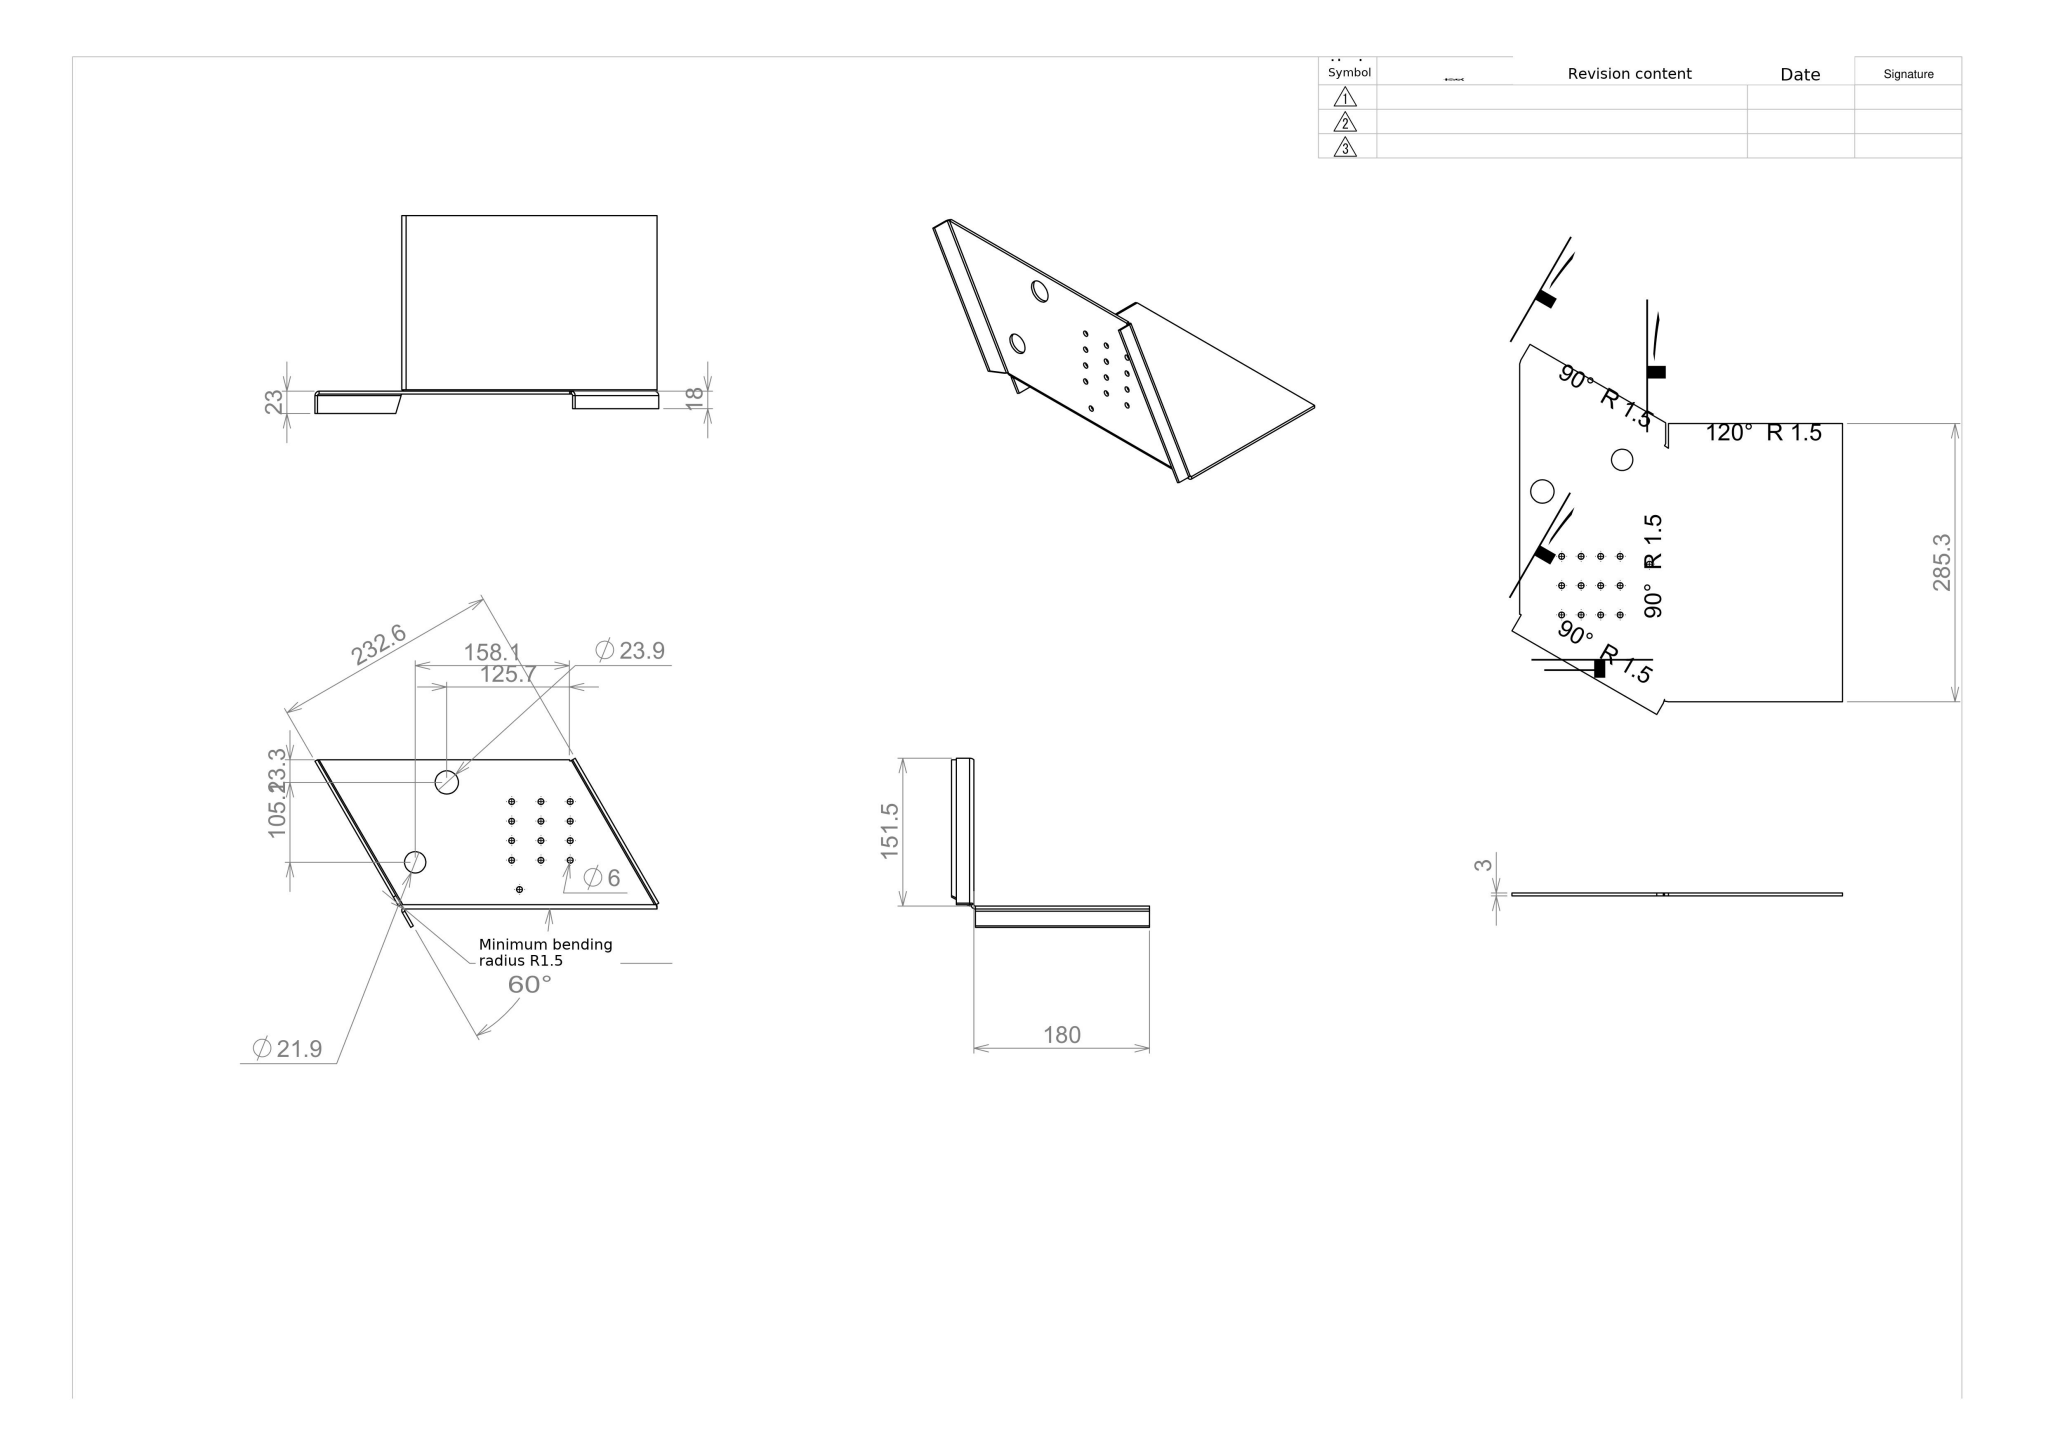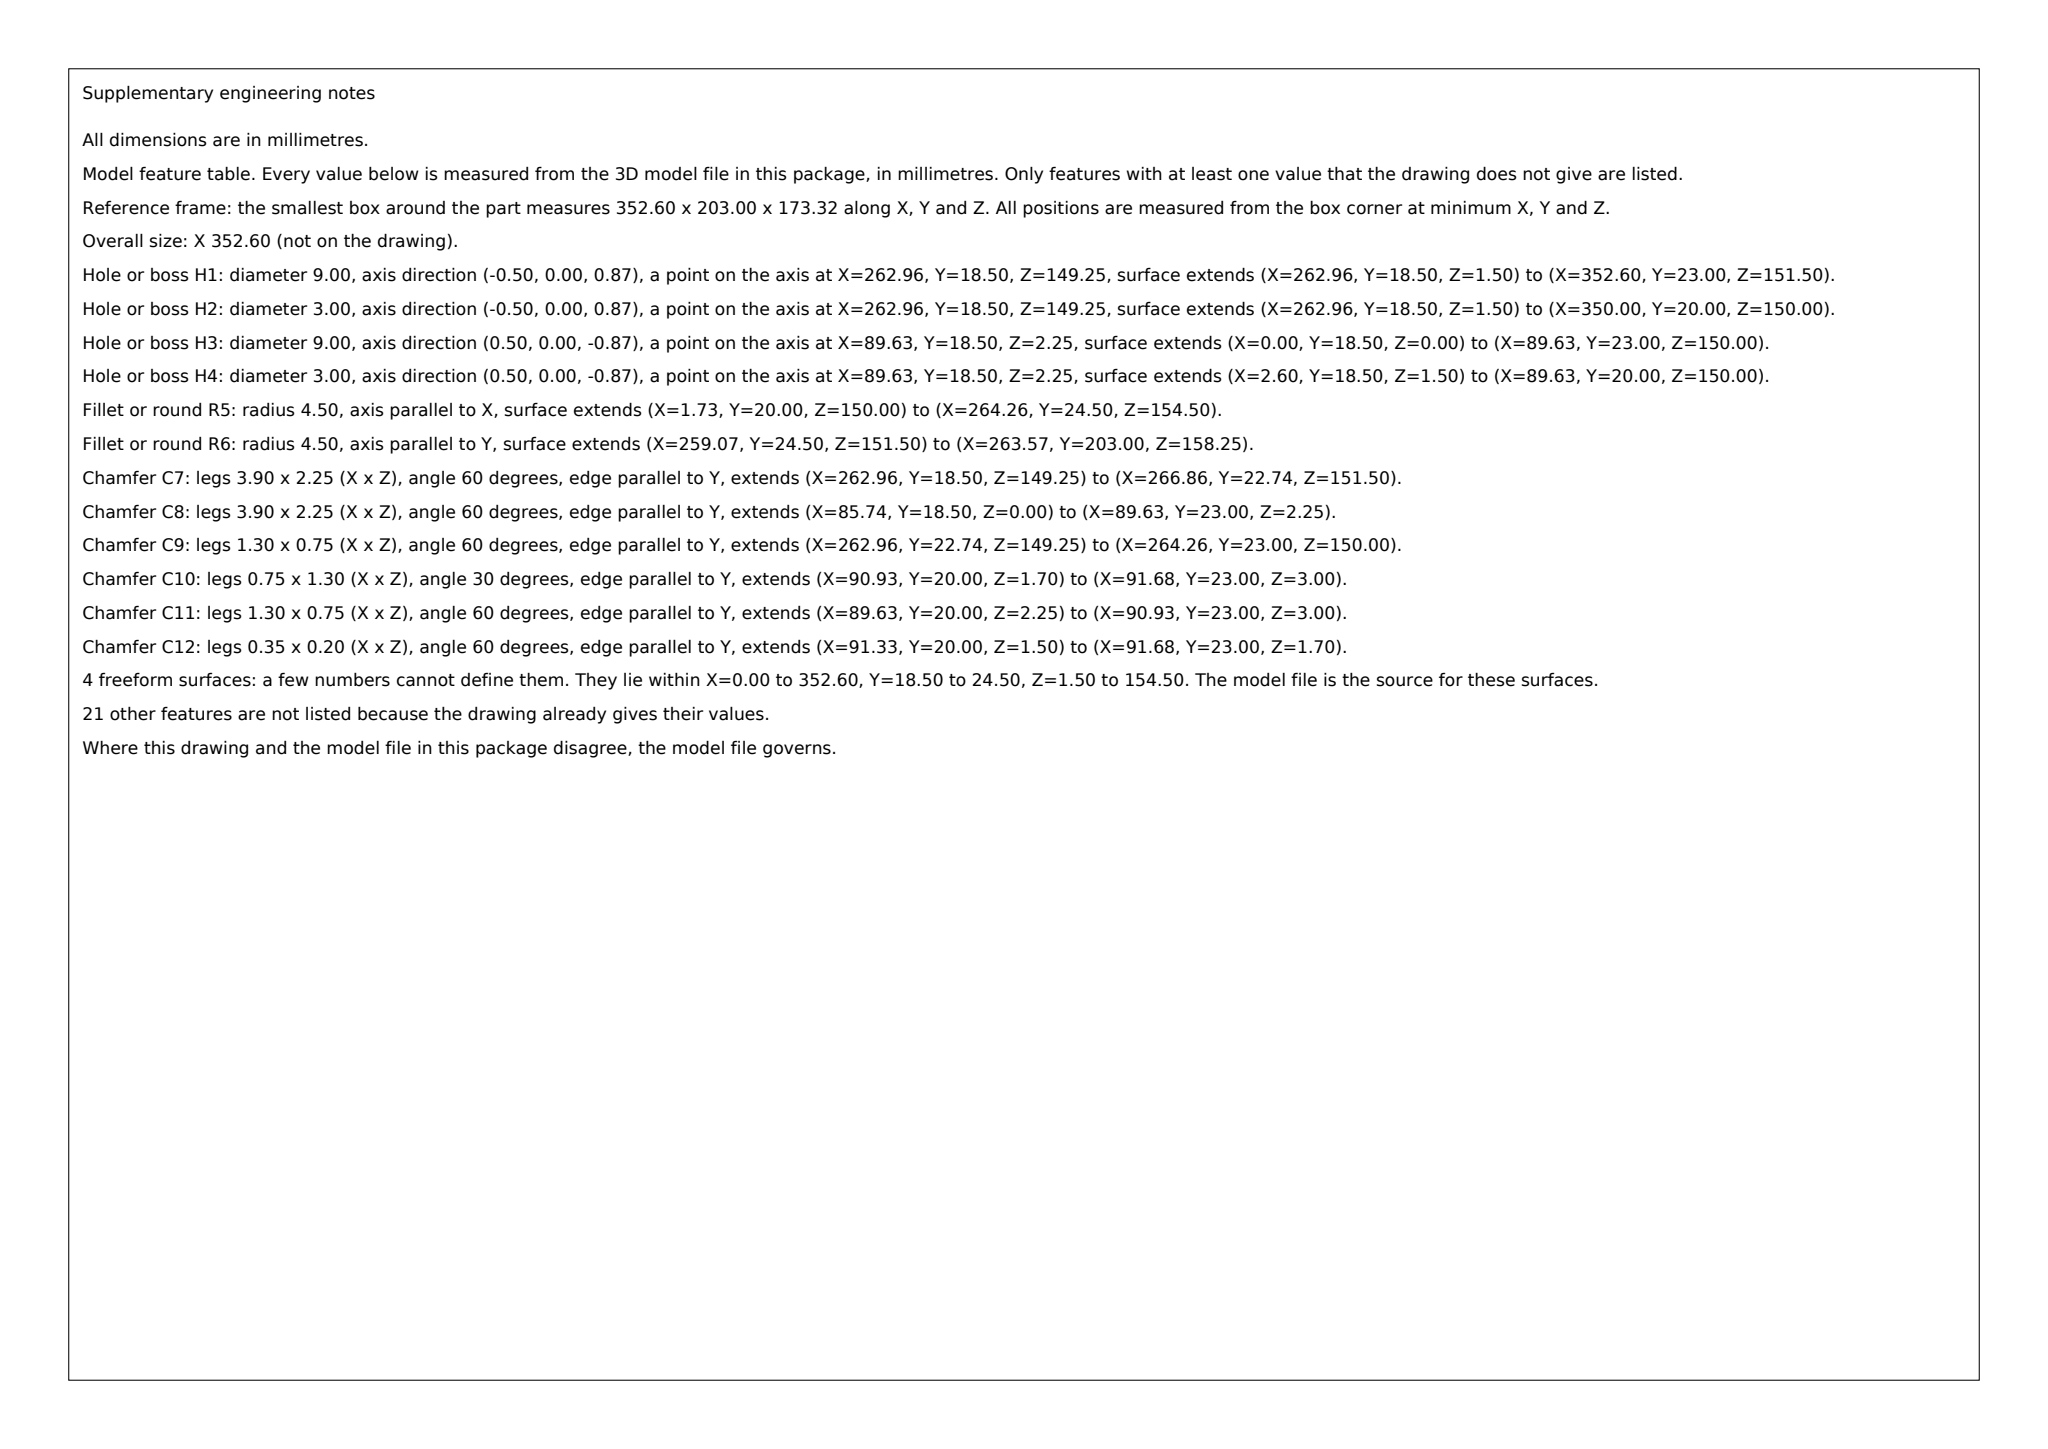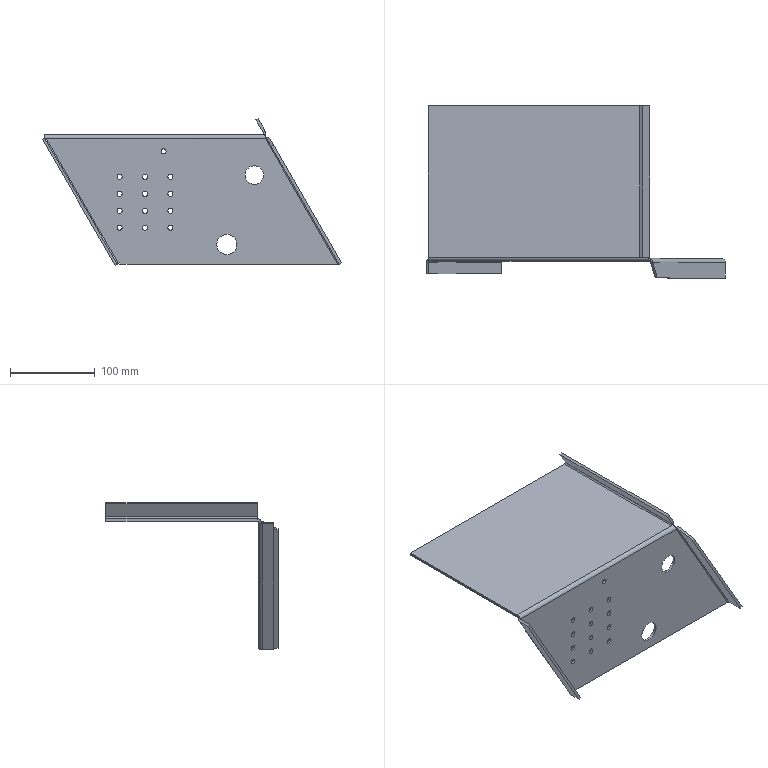Part | SolidWorks | mm | 1 solid | 74 faces | box 352.6 x 203 x 173.32 mm | volume 286620 mm3 | cylinder 38 | plane 32 | spline 4 | commonest cylinder face diameters 6 x26 9 x4 3 x4 23.873 x2 21.908 x2